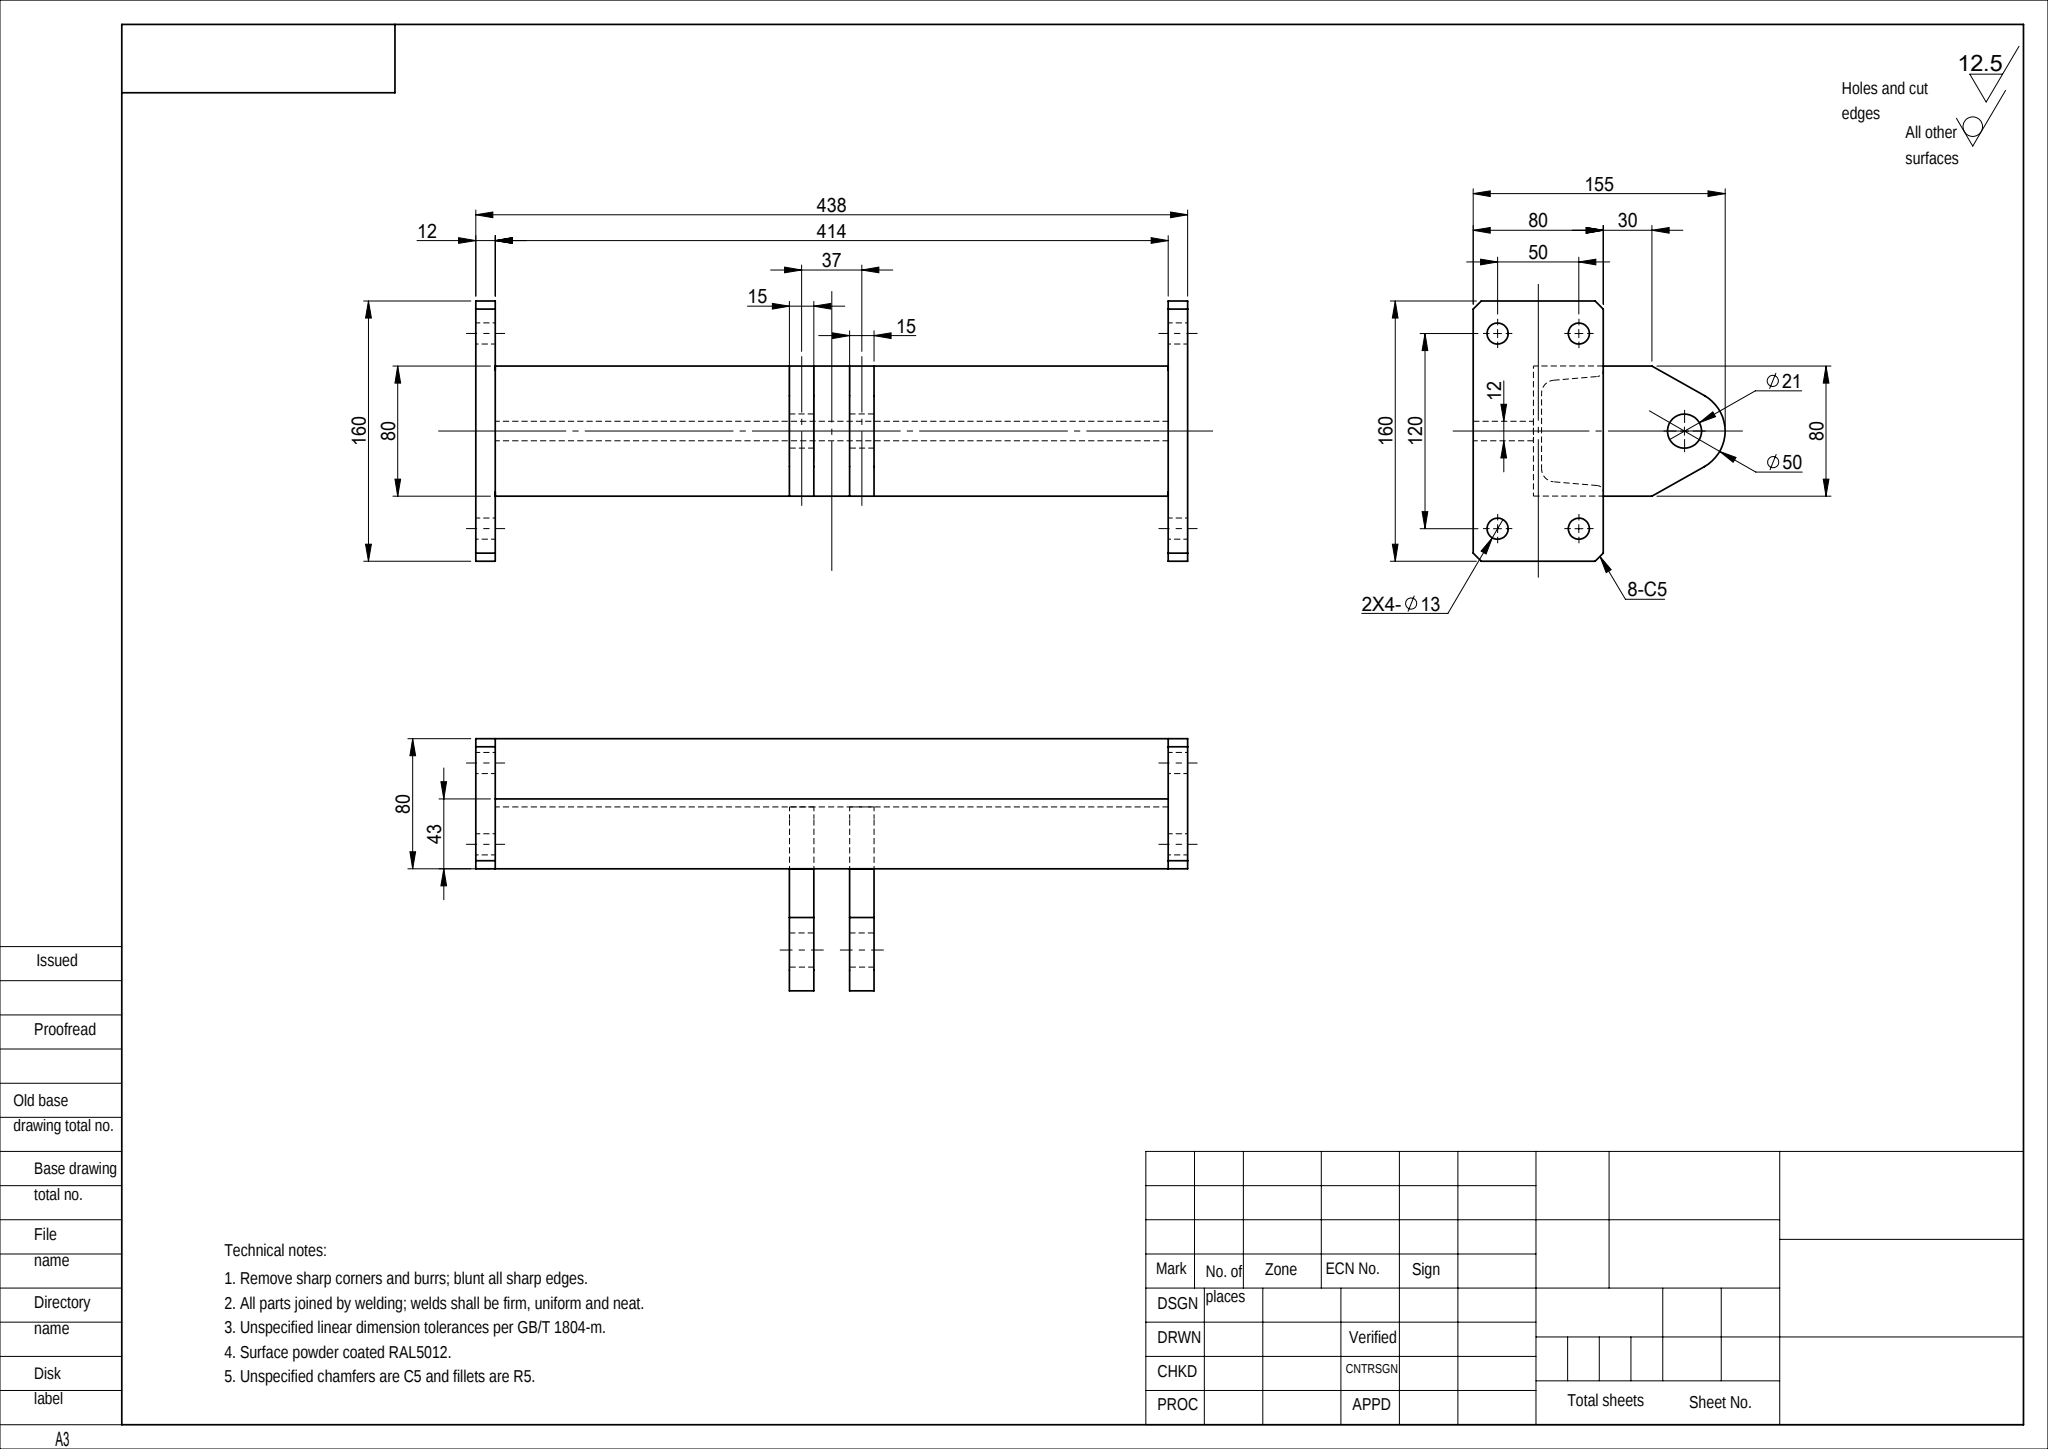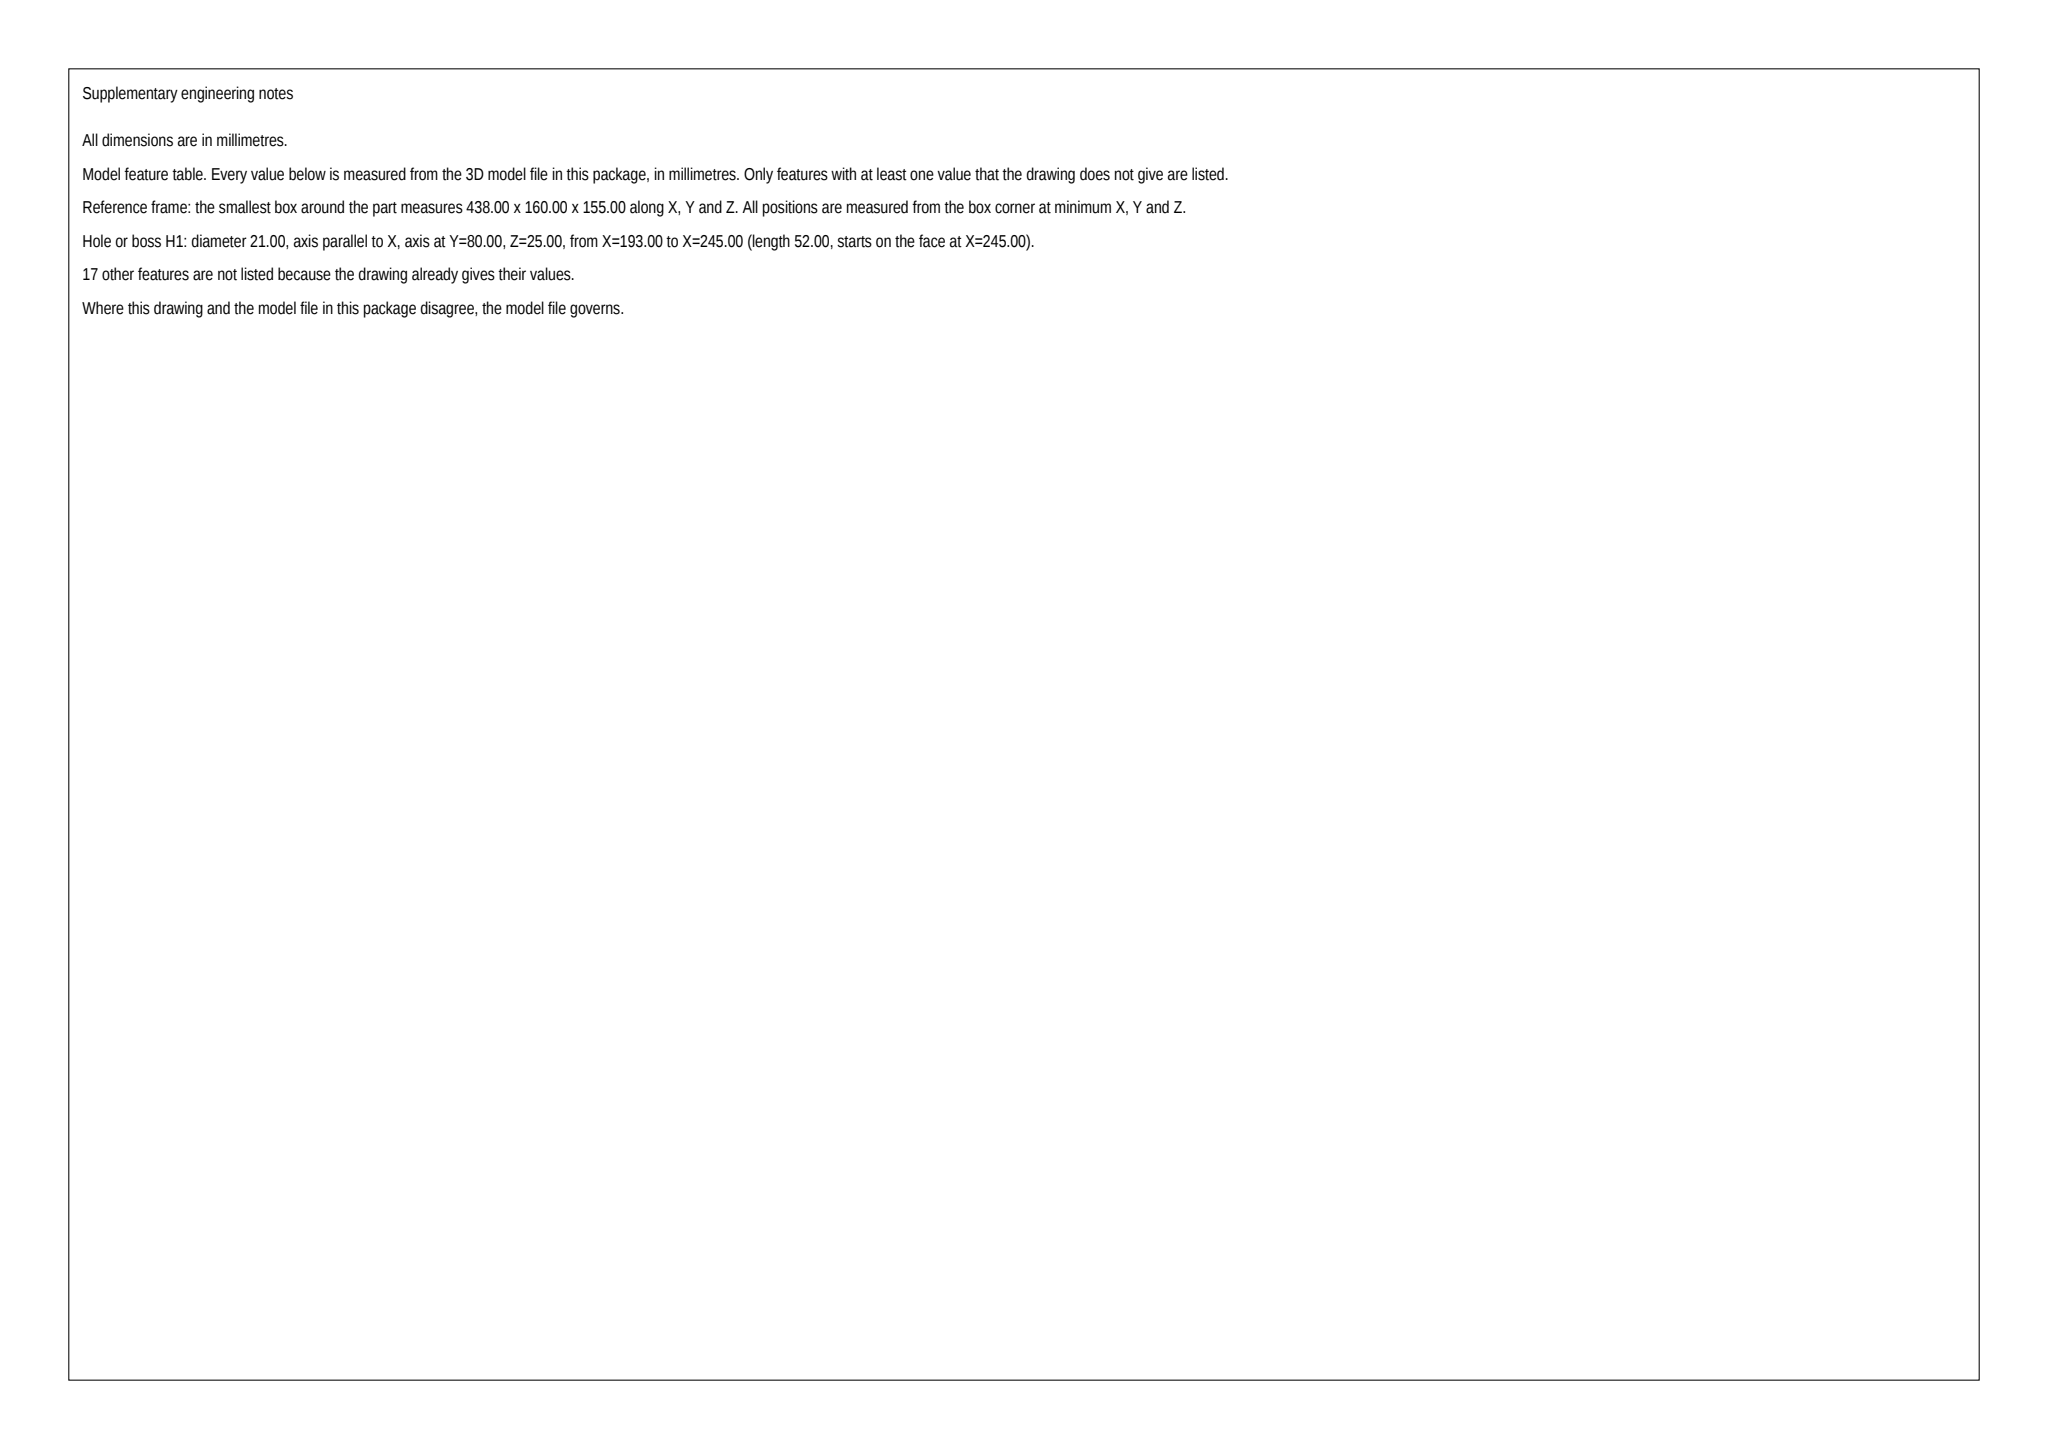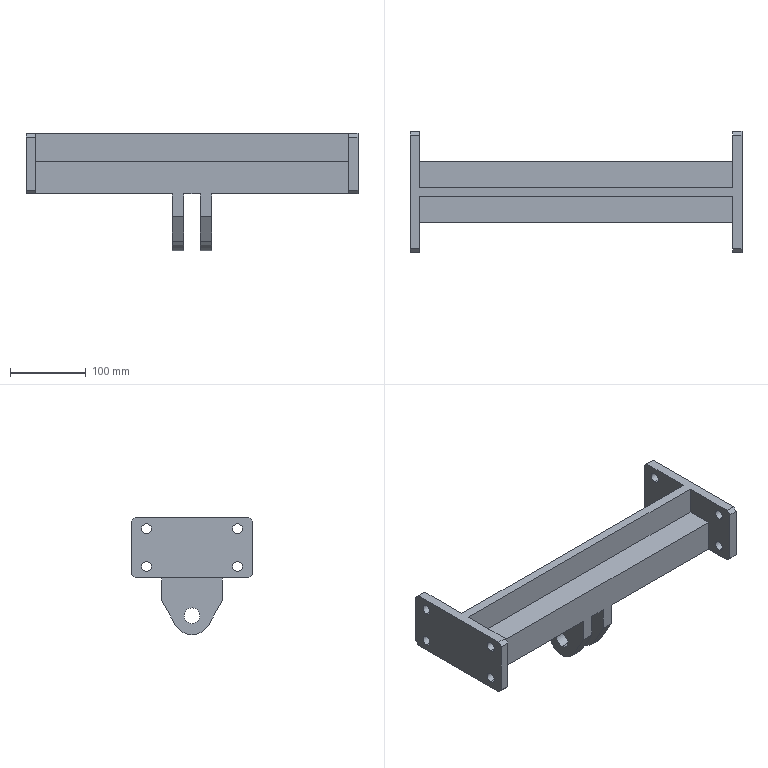Part | SolidWorks | mm | 1 solid | 82 faces | box 438 x 160 x 155 mm | volume 1100807 mm3 | plane 48 | cylinder 34 | commonest cylinder face diameters 13 x16 8 x6 16 x6 21 x4 50 x2
Drawing notes:
SECT CAVITY 414 LG: 75 W AT BTM FACE, 46.4 W AT TOP x 38 DEEP | from the solid: z=75 lips y40-42.5 & 117.5-120 (opening 42.5-117.5=75); z=113 face y56.8-103.2=46.4; cavity 113-75=38; faces x12-426=414
INT FILLETS R8, CTR 23.2 EA SIDE OF SECT CL, 30 ABOVE BTM FACE | from the solid: concave arcs Ø16 axis x at y=56.8/103.2 (CL y=80), z=105 (z-75=30), x12-426
EXT RNDS R4, CTR 37.5 EA SIDE OF SECT CL, 4 ABOVE BTM FACE | from the solid: convex arcs Ø8 axis x at y=42.5/117.5 (CL y=80), z=79 (z-75=4)
CAVITY SIDE WALLS 4.9° FROM VERT, 3.7 TO 30.7 ABOVE BTM FACE | from the solid: inclined planes angle_to_xyz [90,4.9,85.1] bbox_from z=78.7, size z=27 (78.7-105.7); z-75 = 3.7 to 30.7
BTM LIPS 2.5 W EA SIDE; CAVITY ROOF 38 UP, 5 THK TO 43 FACE | from the solid: z=75 faces y40-42.5 & 117.5-120; z=113 roof; z=118 shelf (43 above z=75), 118-113=5
LUG PLATES 15 THK EXTEND 38 INTO BEAM ABOVE BTM FACE | from the solid: lug planes x193/208/230/245, z 0-113, top z=113 vs beam btm z=75 → 38; plate thk 208-193=15
LUG FLANK TAPER 29.4° TO LUG CL, TANG TO Ø50 END R, 4 PL | from the solid: inclined planes angle_to_xyz [90,29.4,60.6] at x193/230, tangent to Ø50 convex arc at y80, z25
build123d program:
from build123d import *

# Parameters (mm, degrees)
GB_T707_1988_HOT_ROLLED_CHANNEL_STEEL_8_DEPTH = 414
SKETCH3_W                                     = 80
SKETCH3_H                                     = 160
BOSS_EXTRUDE1_DEPTH                           = 12
SKETCH5_W                                     = 6.5
SKETCH5_H                                     = 438
F_13_0_13_DIAMETER_HOLE1_AT_2_COUNT           = 2
F_13_0_13_DIAMETER_HOLE1_AT_2_PITCH           = 50
F_13_0_13_DIAMETER_HOLE1_AT_3_COUNT           = 2
F_13_0_13_DIAMETER_HOLE1_AT_3_PITCH           = 130
F_13_0_13_DIAMETER_HOLE1_AT_4_COUNT           = 2
F_13_0_13_DIAMETER_HOLE1_AT_4_PITCH           = 120
CHAMFER1_SIZE                                 = 5
CHAMFER2_SIZE                                 = 5
BOSS_EXTRUDE2_START                           = 18.5
SKETCH6_2_R                                   = 10.5
BOSS_EXTRUDE2_DEPTH                           = 7.5
BOSS_EXTRUDE3_START                           = -18.5
SKETCH6_2_2_R                                 = 10.5
BOSS_EXTRUDE3_DEPTH                           = 7.5
BOSS_EXTRUDE4_REACH                           = 451.222
SKETCH7_W                                     = 37
SKETCH7_H                                     = 12


with BuildPart() as part:
    # Sketch1 → GB_T707-1988 Hot Rolled Channel Steel 8 (new body)
    with BuildSketch(Plane(origin=(-207, -40, 0), x_dir=(0, 0, 1), z_dir=(1, 0, 0))):
        with BuildLine():
            Line((0, 0), (0, -80))
            Line((0, -80), (-43, -80))
            Line((-43, -80), (-43, -77.511))
            ThreePointArc((-43, -77.511), (-41.946, -74.806), (-39.341, -73.526))
            Line((-39.341, -73.526), (-12.318, -71.215))
            ThreePointArc((-12.318, -71.215), (-7.107, -68.654), (-5, -63.244))
            Line((-5, -63.244), (-5, -16.756))
            ThreePointArc((-5, -16.756), (-7.107, -11.346), (-12.318, -8.785))
            Line((-12.318, -8.785), (-39.341, -6.474))
            ThreePointArc((-39.341, -6.474), (-41.946, -5.194), (-43, -2.489))
            Line((-43, -2.489), (-43, 0))
            Line((-43, 0), (0, 0))
        make_face()
    extrude(amount=GB_T707_1988_HOT_ROLLED_CHANNEL_STEEL_8_DEPTH)


with BuildPart() as body_2:
    # Sketch3 → Boss-Extrude1 (new body)
    with BuildSketch(Plane(origin=(207, 0, 0), x_dir=(0, 0, -1), z_dir=(1, 0, 0))):
        with Locations((3, 0)):
            Rectangle(SKETCH3_W, SKETCH3_H)
    extrude(amount=BOSS_EXTRUDE1_DEPTH)


with BuildPart() as body_3:
    # Mirror1: mirrored copy
    add(body_2.part.mirror(Plane(origin=(0, 0, 0), x_dir=(0, 0, 1), z_dir=(1, 0, 0))))


with BuildPart() as f_13_0_13_diameter_hole1_tool:
    # Sketch5 → 13.0 _13_ Diameter Hole1 (revolve)
    with BuildSketch(Plane(origin=(219, 60, 22), x_dir=(0, 0, -1), z_dir=(0, 1, 0))):
        with Locations((3.25, 219)):
            Rectangle(SKETCH5_W, SKETCH5_H)
    f_13_0_13_diameter_hole1 = revolve(axis=Axis((225.35, 60, 22), (-1, 0, 0)))


with BuildPart() as body_2_1:
    add(body_2.part)

    # 13.0 _13_ Diameter Hole1: cut by f_13_0_13_diameter_hole1_tool
    add(f_13_0_13_diameter_hole1_tool.part, mode=Mode.SUBTRACT)


with BuildPart() as body_3_1:
    add(body_3.part)

    # 13.0 _13_ Diameter Hole1: cut by f_13_0_13_diameter_hole1_tool
    add(f_13_0_13_diameter_hole1_tool.part, mode=Mode.SUBTRACT)


with BuildPart() as f_13_0_13_diameter_hole1_at_2_tool:
    # 13.0 _13_ Diameter Hole1 at 2: 13.0 _13_ Diameter Hole1 ×2
    with Locations(*[(0, 0, -i * F_13_0_13_DIAMETER_HOLE1_AT_2_PITCH) for i in range(1, F_13_0_13_DIAMETER_HOLE1_AT_2_COUNT)]):
        add(f_13_0_13_diameter_hole1)


with BuildPart() as body_2_2:
    add(body_2_1.part)

    # 13.0 _13_ Diameter Hole1 at 2: cut by f_13_0_13_diameter_hole1_at_2_tool
    add(f_13_0_13_diameter_hole1_at_2_tool.part, mode=Mode.SUBTRACT)


with BuildPart() as body_3_2:
    add(body_3_1.part)

    # 13.0 _13_ Diameter Hole1 at 2: cut by f_13_0_13_diameter_hole1_at_2_tool
    add(f_13_0_13_diameter_hole1_at_2_tool.part, mode=Mode.SUBTRACT)


with BuildPart() as f_13_0_13_diameter_hole1_at_3_tool:
    # 13.0 _13_ Diameter Hole1 at 3: 13.0 _13_ Diameter Hole1 ×2
    with Locations(*[Vector(0, -0.9231, -0.3846) * (i * F_13_0_13_DIAMETER_HOLE1_AT_3_PITCH) for i in range(1, F_13_0_13_DIAMETER_HOLE1_AT_3_COUNT)]):
        add(f_13_0_13_diameter_hole1)


with BuildPart() as body_2_3:
    add(body_2_2.part)

    # 13.0 _13_ Diameter Hole1 at 3: cut by f_13_0_13_diameter_hole1_at_3_tool
    add(f_13_0_13_diameter_hole1_at_3_tool.part, mode=Mode.SUBTRACT)


with BuildPart() as body_3_3:
    add(body_3_2.part)

    # 13.0 _13_ Diameter Hole1 at 3: cut by f_13_0_13_diameter_hole1_at_3_tool
    add(f_13_0_13_diameter_hole1_at_3_tool.part, mode=Mode.SUBTRACT)


with BuildPart() as f_13_0_13_diameter_hole1_at_4_tool:
    # 13.0 _13_ Diameter Hole1 at 4: 13.0 _13_ Diameter Hole1 ×2
    with Locations(*[(0, -i * F_13_0_13_DIAMETER_HOLE1_AT_4_PITCH, 0) for i in range(1, F_13_0_13_DIAMETER_HOLE1_AT_4_COUNT)]):
        add(f_13_0_13_diameter_hole1)


with BuildPart() as body_2_4:
    add(body_2_3.part)

    # 13.0 _13_ Diameter Hole1 at 4: cut by f_13_0_13_diameter_hole1_at_4_tool
    add(f_13_0_13_diameter_hole1_at_4_tool.part, mode=Mode.SUBTRACT)

    # Chamfer2
    chamfer2_edges = [body_2_4.edges().sort_by_distance(p)[0] for p in [
        (213, 80, 37),
        (213, 80, -43),
        (213, -80, -43),
        (213, -80, 37),
    ]]
    chamfer(chamfer2_edges, length=CHAMFER2_SIZE)


with BuildPart() as body_3_4:
    add(body_3_3.part)

    # 13.0 _13_ Diameter Hole1 at 4: cut by f_13_0_13_diameter_hole1_at_4_tool
    add(f_13_0_13_diameter_hole1_at_4_tool.part, mode=Mode.SUBTRACT)

    # Chamfer1
    chamfer1_edges = [body_3_4.edges().sort_by_distance(p)[0] for p in [
        (-213, 80, 37),
        (-213, 80, -43),
        (-213, -80, -43),
        (-213, -80, 37),
    ]]
    chamfer(chamfer1_edges, length=CHAMFER1_SIZE)


with BuildPart() as body_4:
    # Sketch6_2 → Boss-Extrude2 (new, symmetric)
    with BuildSketch(Plane(origin=(0, 0, 0), x_dir=(0, 0, -1), z_dir=(1, 0, 0)).offset(BOSS_EXTRUDE2_START)):
        with BuildLine():
            Line((43, 40), (73, 40))
            Line((73, 40), (105.29, 21.77))
            ThreePointArc((105.29, 21.77), (118, 0), (105.29, -21.77))
            Line((105.29, -21.77), (73, -40))
            Line((73, -40), (43, -40))
            Line((43, -40), (43, -37.511))
            ThreePointArc((43, -37.511), (41.946, -34.806), (39.341, -33.526))
            Line((39.341, -33.526), (12.318, -31.215))
            ThreePointArc((12.318, -31.215), (7.107, -28.654), (5, -23.244))
            Line((5, -23.244), (5, 23.244))
            ThreePointArc((5, 23.244), (7.107, 28.654), (12.318, 31.215))
            Line((12.318, 31.215), (39.341, 33.526))
            ThreePointArc((39.341, 33.526), (41.946, 34.806), (43, 37.511))
            Line((43, 37.511), (43, 40))
        make_face()
        with Locations((93, 0)):
            Circle(SKETCH6_2_R, mode=Mode.SUBTRACT)
    extrude(amount=BOSS_EXTRUDE2_DEPTH, both=True)


with BuildPart() as body_5:
    # Sketch6_2 2 → Boss-Extrude3 (new, symmetric)
    with BuildSketch(Plane(origin=(0, 0, 0), x_dir=(0, 0, -1), z_dir=(1, 0, 0)).offset(BOSS_EXTRUDE3_START)):
        with BuildLine():
            Line((43, 40), (73, 40))
            Line((73, 40), (105.29, 21.77))
            ThreePointArc((105.29, 21.77), (118, 0), (105.29, -21.77))
            Line((105.29, -21.77), (73, -40))
            Line((73, -40), (43, -40))
            Line((43, -40), (43, -37.511))
            ThreePointArc((43, -37.511), (41.946, -34.806), (39.341, -33.526))
            Line((39.341, -33.526), (12.318, -31.215))
            ThreePointArc((12.318, -31.215), (7.107, -28.654), (5, -23.244))
            Line((5, -23.244), (5, 23.244))
            ThreePointArc((5, 23.244), (7.107, 28.654), (12.318, 31.215))
            Line((12.318, 31.215), (39.341, 33.526))
            ThreePointArc((39.341, 33.526), (41.946, 34.806), (43, 37.511))
            Line((43, 37.511), (43, 40))
        make_face()
        with Locations((93, 0)):
            Circle(SKETCH6_2_2_R, mode=Mode.SUBTRACT)
    extrude(amount=BOSS_EXTRUDE3_DEPTH, both=True)


with BuildPart() as body_6:

    # Sketch7 → Boss-Extrude4 (new, up to next)
    with BuildSketch(Plane(origin=(-207, 0, 0), x_dir=(0, 0, -1), z_dir=(1, 0, 0)), mode=Mode.PRIVATE) as boss_extrude4_sk1:
        with Locations((-18.5, 0)):
            Rectangle(SKETCH7_W, SKETCH7_H)
    boss_extrude4_tool1 = extrude(boss_extrude4_sk1.sketch, amount=BOSS_EXTRUDE4_REACH, mode=Mode.PRIVATE) - body_2_4.part
    add(boss_extrude4_tool1.solids().sort_by_distance((-207, 0, 18.5))[0])


with BuildPart() as body_4_1:
    add(body_4.part)

    # Combine-RayDong-Repair: union body 2, body 6, body 5, part, body 3
    add(body_2_4.part)
    add(body_6.part)
    add(body_5.part)
    add(part.part)
    add(body_3_4.part)


solid = body_4_1.part